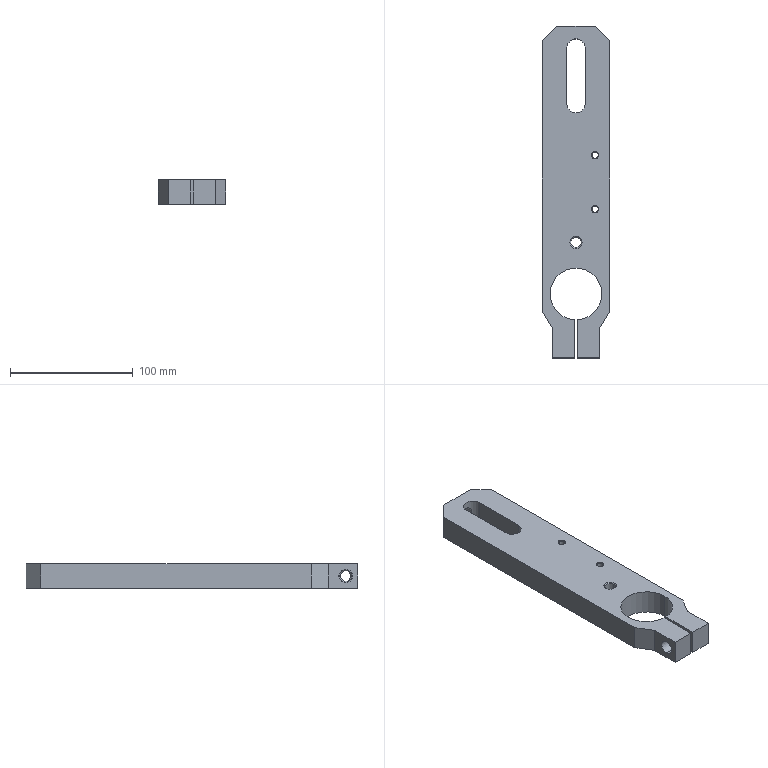Component | SolidWorks | DoubleFilmTransport-1_WheelTensionAdjustmentPlate-1 | 1 solid | 42 faces | box 55 x 270 x 20 mm | volume 232232 mm3 | cylinder 17 | plane 17 | cone 8 | commonest cylinder face diameters 8.5 x4 5 x4 42 x3 11 x2 9 x2 15 x2
build123d program:
from build123d import *

# Parameters (mm, degrees)
BOSS_EXTRUDE1_DEPTH                                  = 20
CUT_EXTRUDE1_DEPTH                                   = 221.636
CUT_EXTRUDE2_DEPTH                                   = 221.636
CUT_EXTRUDE3_DEPTH                                   = 221.636
CUT_EXTRUDE4_DEPTH                                   = 221.636
SKETCH6_W                                            = 21
SKETCH6_H                                            = 20
COUNTERSUNK_HOLE_1_FOR_M8_FLAT_HEAD_MACH_D           = 8.5
COUNTERSUNK_HOLE_1_FOR_M8_FLAT_HEAD_MACH_CSINK_D     = 10.05
COUNTERSUNK_HOLE_1_FOR_M8_FLAT_HEAD_MACH_CSINK_ANGLE = 90
F_5_0_5_DIAMETER_HOLE1_D                             = 5
F_5_0_5_DIAMETER_HOLE1_CSINK_D                       = 6.05
F_5_0_5_DIAMETER_HOLE1_CSINK_ANGLE                   = 90
F_9_0_9_DIAMETER_HOLE1_REACH                         = 273.581
F_9_0_9_DIAMETER_HOLE1_BORE_R                        = 4.5
SKETCH15_W                                           = 5.5
SKETCH15_H                                           = 26.5


with BuildPart() as part:
    # Sketch1 → Boss-Extrude1 (new body)
    with BuildSketch(Plane.XY.offset(10)):
        Polygon((-27.5, 206), (-27.5, -52), (27.5, -52), (27.5, 206), (15.5, 218), (-15.5, 218), align=None)
    extrude(amount=-BOSS_EXTRUDE1_DEPTH)

    # Sketch2 → Cut-Extrude1 (cut, through all)
    with BuildSketch(Plane(origin=(0, 0, -10), x_dir=(-1, 0, 0), z_dir=(0, 0, -1))):
        Polygon((27.5, -14), (19, -28), (19, -52), (27.5, -52), align=None)
    extrude(amount=-CUT_EXTRUDE1_DEPTH, mode=Mode.SUBTRACT)

    # Sketch3 → Cut-Extrude2 (cut, through all)
    with BuildSketch(Plane(origin=(0, 0, -10), x_dir=(-1, 0, 0), z_dir=(0, 0, -1))):
        with BuildLine():
            Line((1, -52), (1, -20.976))
            ThreePointArc((1, -20.976), (0, -21), (-1, -20.976))
            Line((-1, -20.976), (-1, -52))
            Line((-1, -52), (1, -52))
        make_face()
    extrude(amount=-CUT_EXTRUDE2_DEPTH, mode=Mode.SUBTRACT)

    # Sketch4 → Cut-Extrude3 (cut, through all)
    with BuildSketch(Plane(origin=(0, 0, -10), x_dir=(-1, 0, 0), z_dir=(0, 0, -1))):
        Polygon((-19, -52), (-19, -28), (-27.5, -14), (-27.5, -52), align=None)
    extrude(amount=-CUT_EXTRUDE3_DEPTH, mode=Mode.SUBTRACT)

    # Sketch5 → Cut-Extrude4 (cut, through all)
    with BuildSketch(Plane(origin=(0, 0, -10), x_dir=(-1, 0, 0), z_dir=(0, 0, -1))):
        with BuildLine():
            Line((7.5, 155), (7.5, 200))
            ThreePointArc((7.5, 200), (0, 207.5), (-7.5, 200))
            Line((-7.5, 200), (-7.5, 155))
            ThreePointArc((-7.5, 155), (0, 147.5), (7.5, 155))
        make_face()
    extrude(amount=-CUT_EXTRUDE4_DEPTH, mode=Mode.SUBTRACT)

    # Sketch6 → Cut-Revolve1 (revolve, cut)
    with BuildSketch(Plane.XZ):
        with Locations((10.5, 0)):
            Rectangle(SKETCH6_W, SKETCH6_H)
    revolve(axis=Axis((0, 0, 10), (0, 0, -1)), mode=Mode.SUBTRACT)

    # Countersunk Hole 1 for M8 Flat Head Mach (through all)
    with Locations(Plane.XY.offset(10)):
        with Locations((0, 42)):
            CounterSinkHole(COUNTERSUNK_HOLE_1_FOR_M8_FLAT_HEAD_MACH_D / 2, COUNTERSUNK_HOLE_1_FOR_M8_FLAT_HEAD_MACH_CSINK_D / 2, counter_sink_angle=COUNTERSUNK_HOLE_1_FOR_M8_FLAT_HEAD_MACH_CSINK_ANGLE)

    # 5.0 _5_ Diameter Hole1 (through all)
    with Locations(Plane.XY.offset(10)):
        with Locations((15.5, 69), (15.5, 113)):
            CounterSinkHole(F_5_0_5_DIAMETER_HOLE1_D / 2, F_5_0_5_DIAMETER_HOLE1_CSINK_D / 2, counter_sink_angle=F_5_0_5_DIAMETER_HOLE1_CSINK_ANGLE)

    # 9.0 _9_ Diameter Hole1 bore → 9.0 _9_ Diameter Hole1 (cut, up to next)
    with BuildSketch(Plane(origin=(0, 218, 0), x_dir=(1, 0, 0), z_dir=(0, 1, 0)), mode=Mode.PRIVATE) as f_9_0_9_diameter_hole1_sk1:
        Circle(F_9_0_9_DIAMETER_HOLE1_BORE_R)
    f_9_0_9_diameter_hole1_tool1 = extrude(f_9_0_9_diameter_hole1_sk1.sketch, amount=-F_9_0_9_DIAMETER_HOLE1_REACH, mode=Mode.PRIVATE) & part.part
    add(f_9_0_9_diameter_hole1_tool1.solids().sort_by_distance((0, 218, 0))[0], mode=Mode.SUBTRACT)

    # Sketch13 → Countersunk Hole 2 for M8 Flat Head Mach (revolve, cut)
    with BuildSketch(Plane(origin=(1, -42, 0), x_dir=(0, 0, 1), z_dir=(0, 1, 0))):
        Polygon((0, 0), (0, 26.5), (4.25, 26.5), (4.25, 0.775), (5.025, 0), align=None)
    revolve(axis=Axis((-5.35, -42, 0), (1, 0, 0)), mode=Mode.SUBTRACT)

    # Sketch15 → 11.0 _11_ Diameter Hole1 (revolve, cut)
    with BuildSketch(Plane(origin=(-1, -42, 0), x_dir=(0, 0, -1), z_dir=(0, 1, 0))):
        with Locations((2.75, 13.25)):
            Rectangle(SKETCH15_W, SKETCH15_H)
    revolve(axis=Axis((5.35, -42, 0), (-1, 0, 0)), mode=Mode.SUBTRACT)


solid = part.part

# Placed as in the assembly
solid = solid.moved(Location((-384.677, 83.374, 86), (0, 0, 0)))